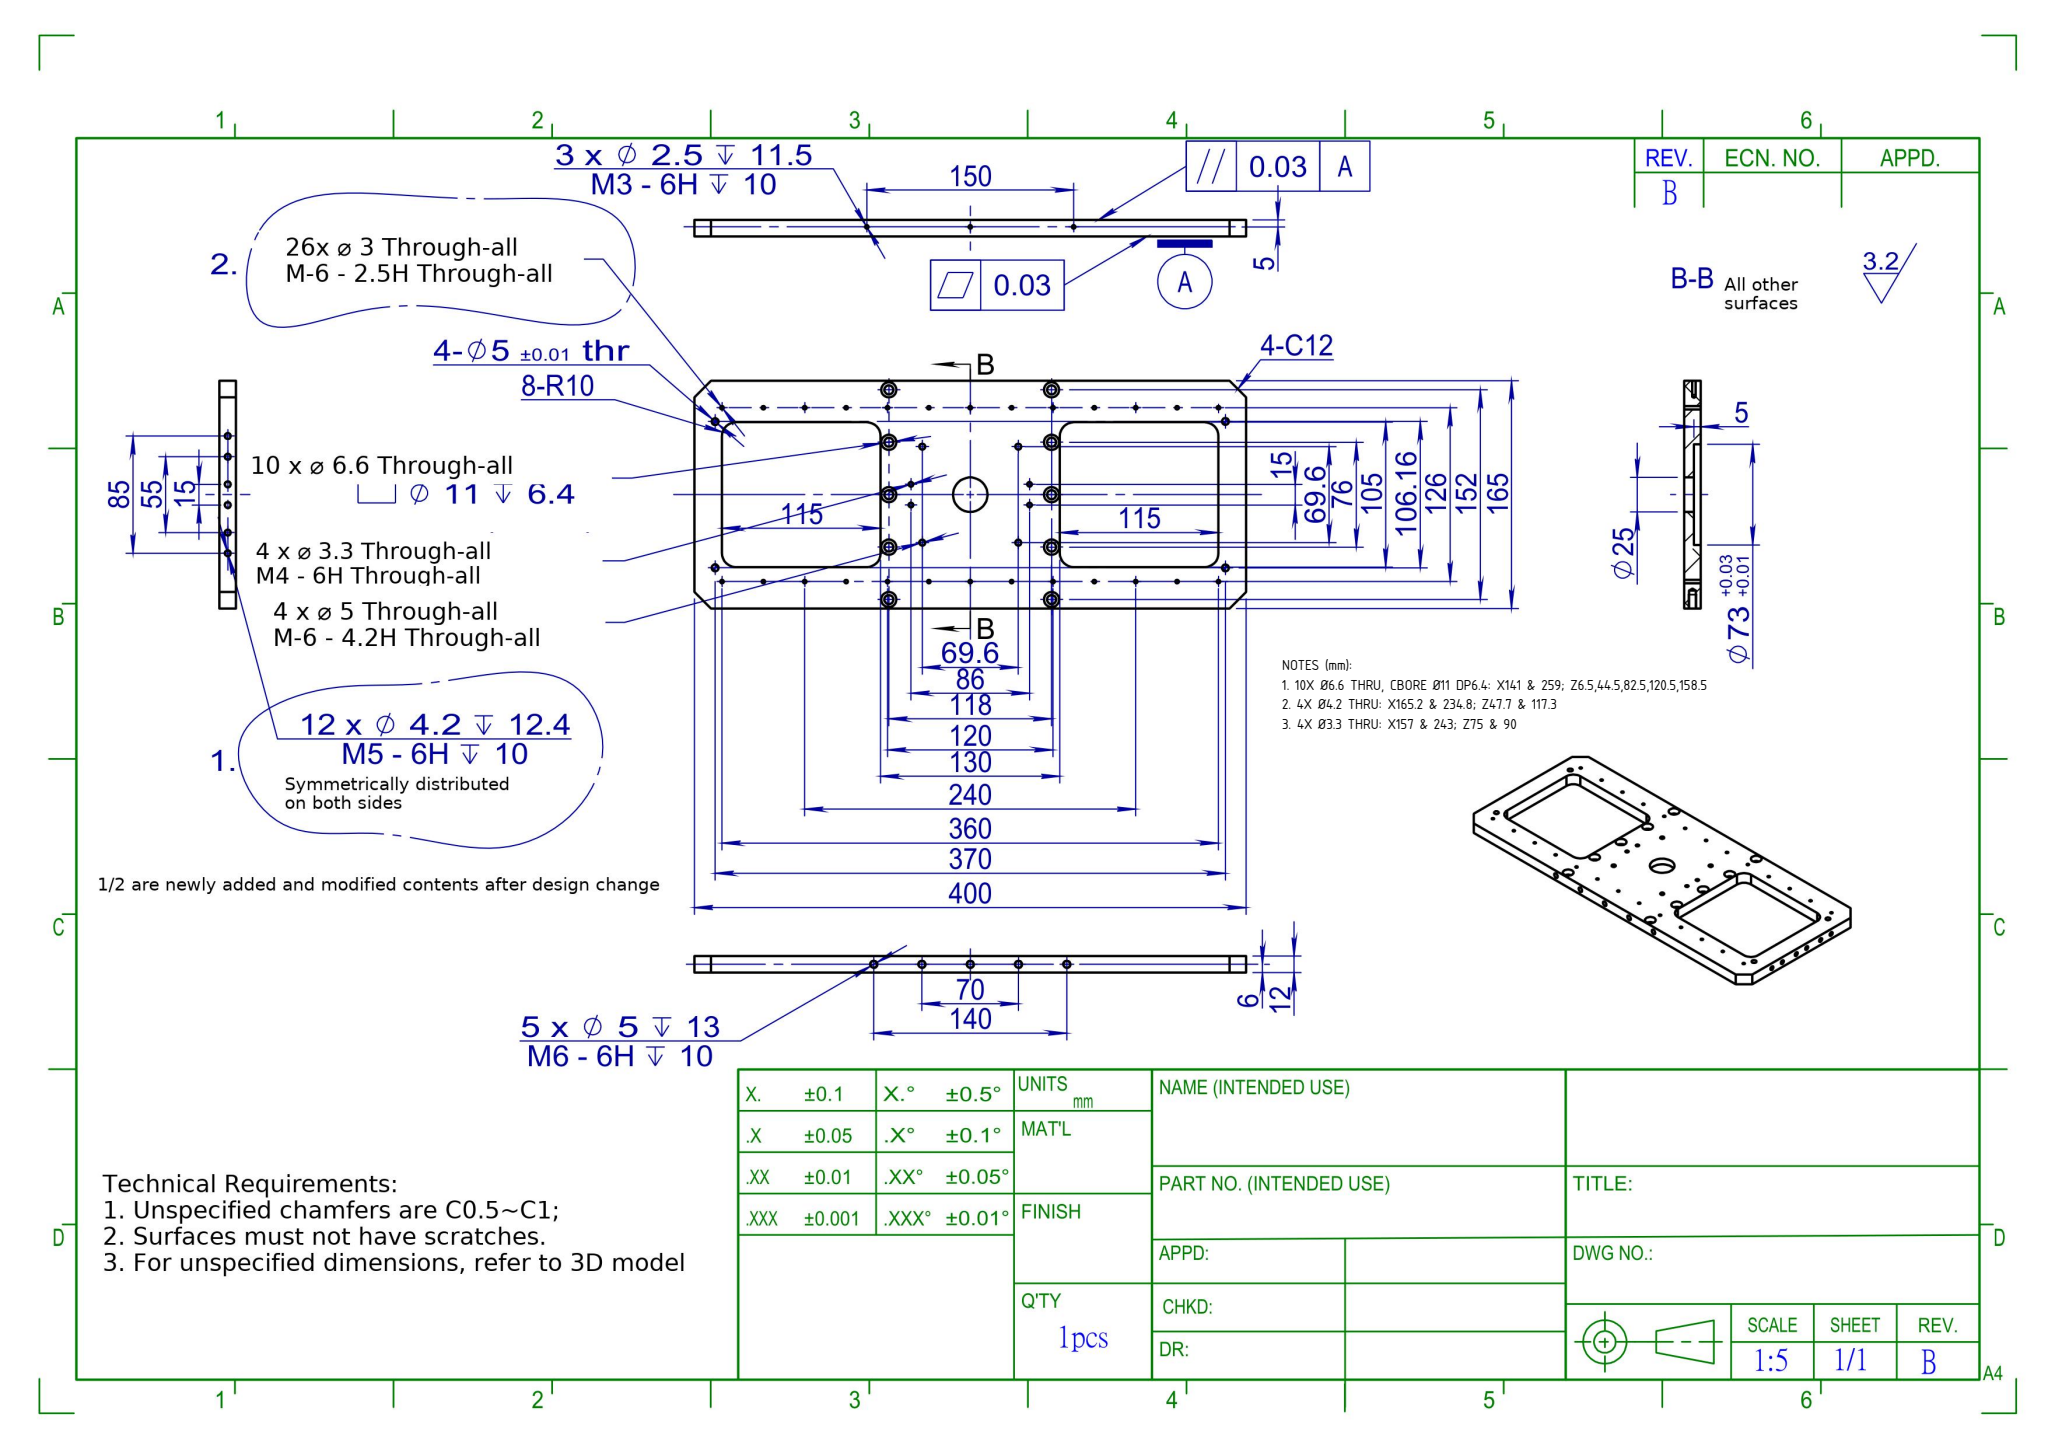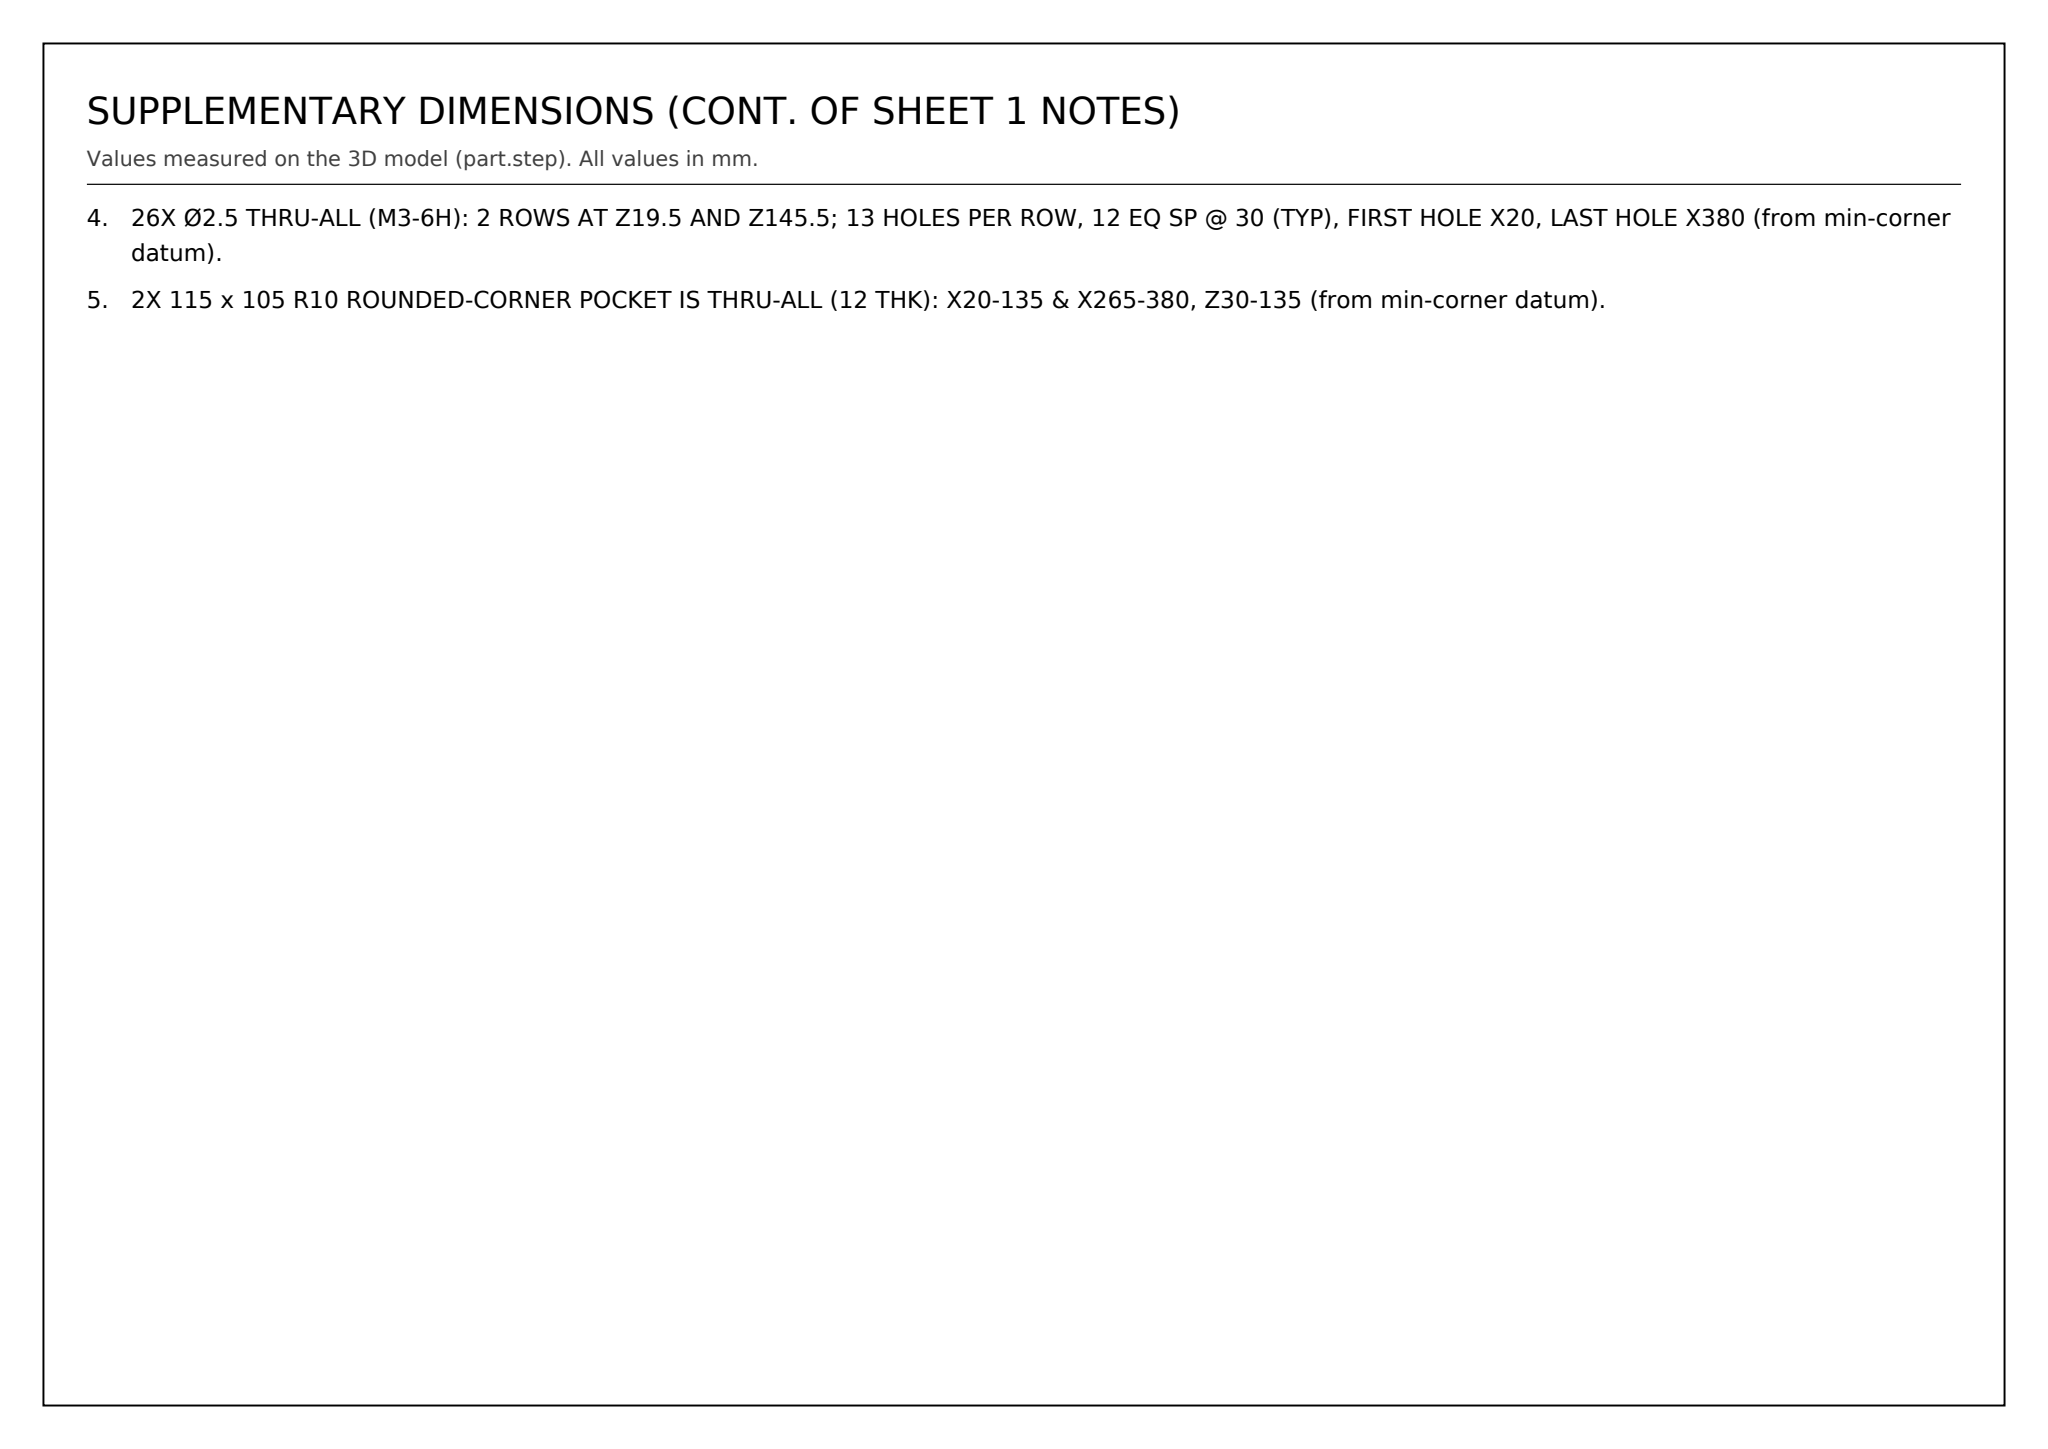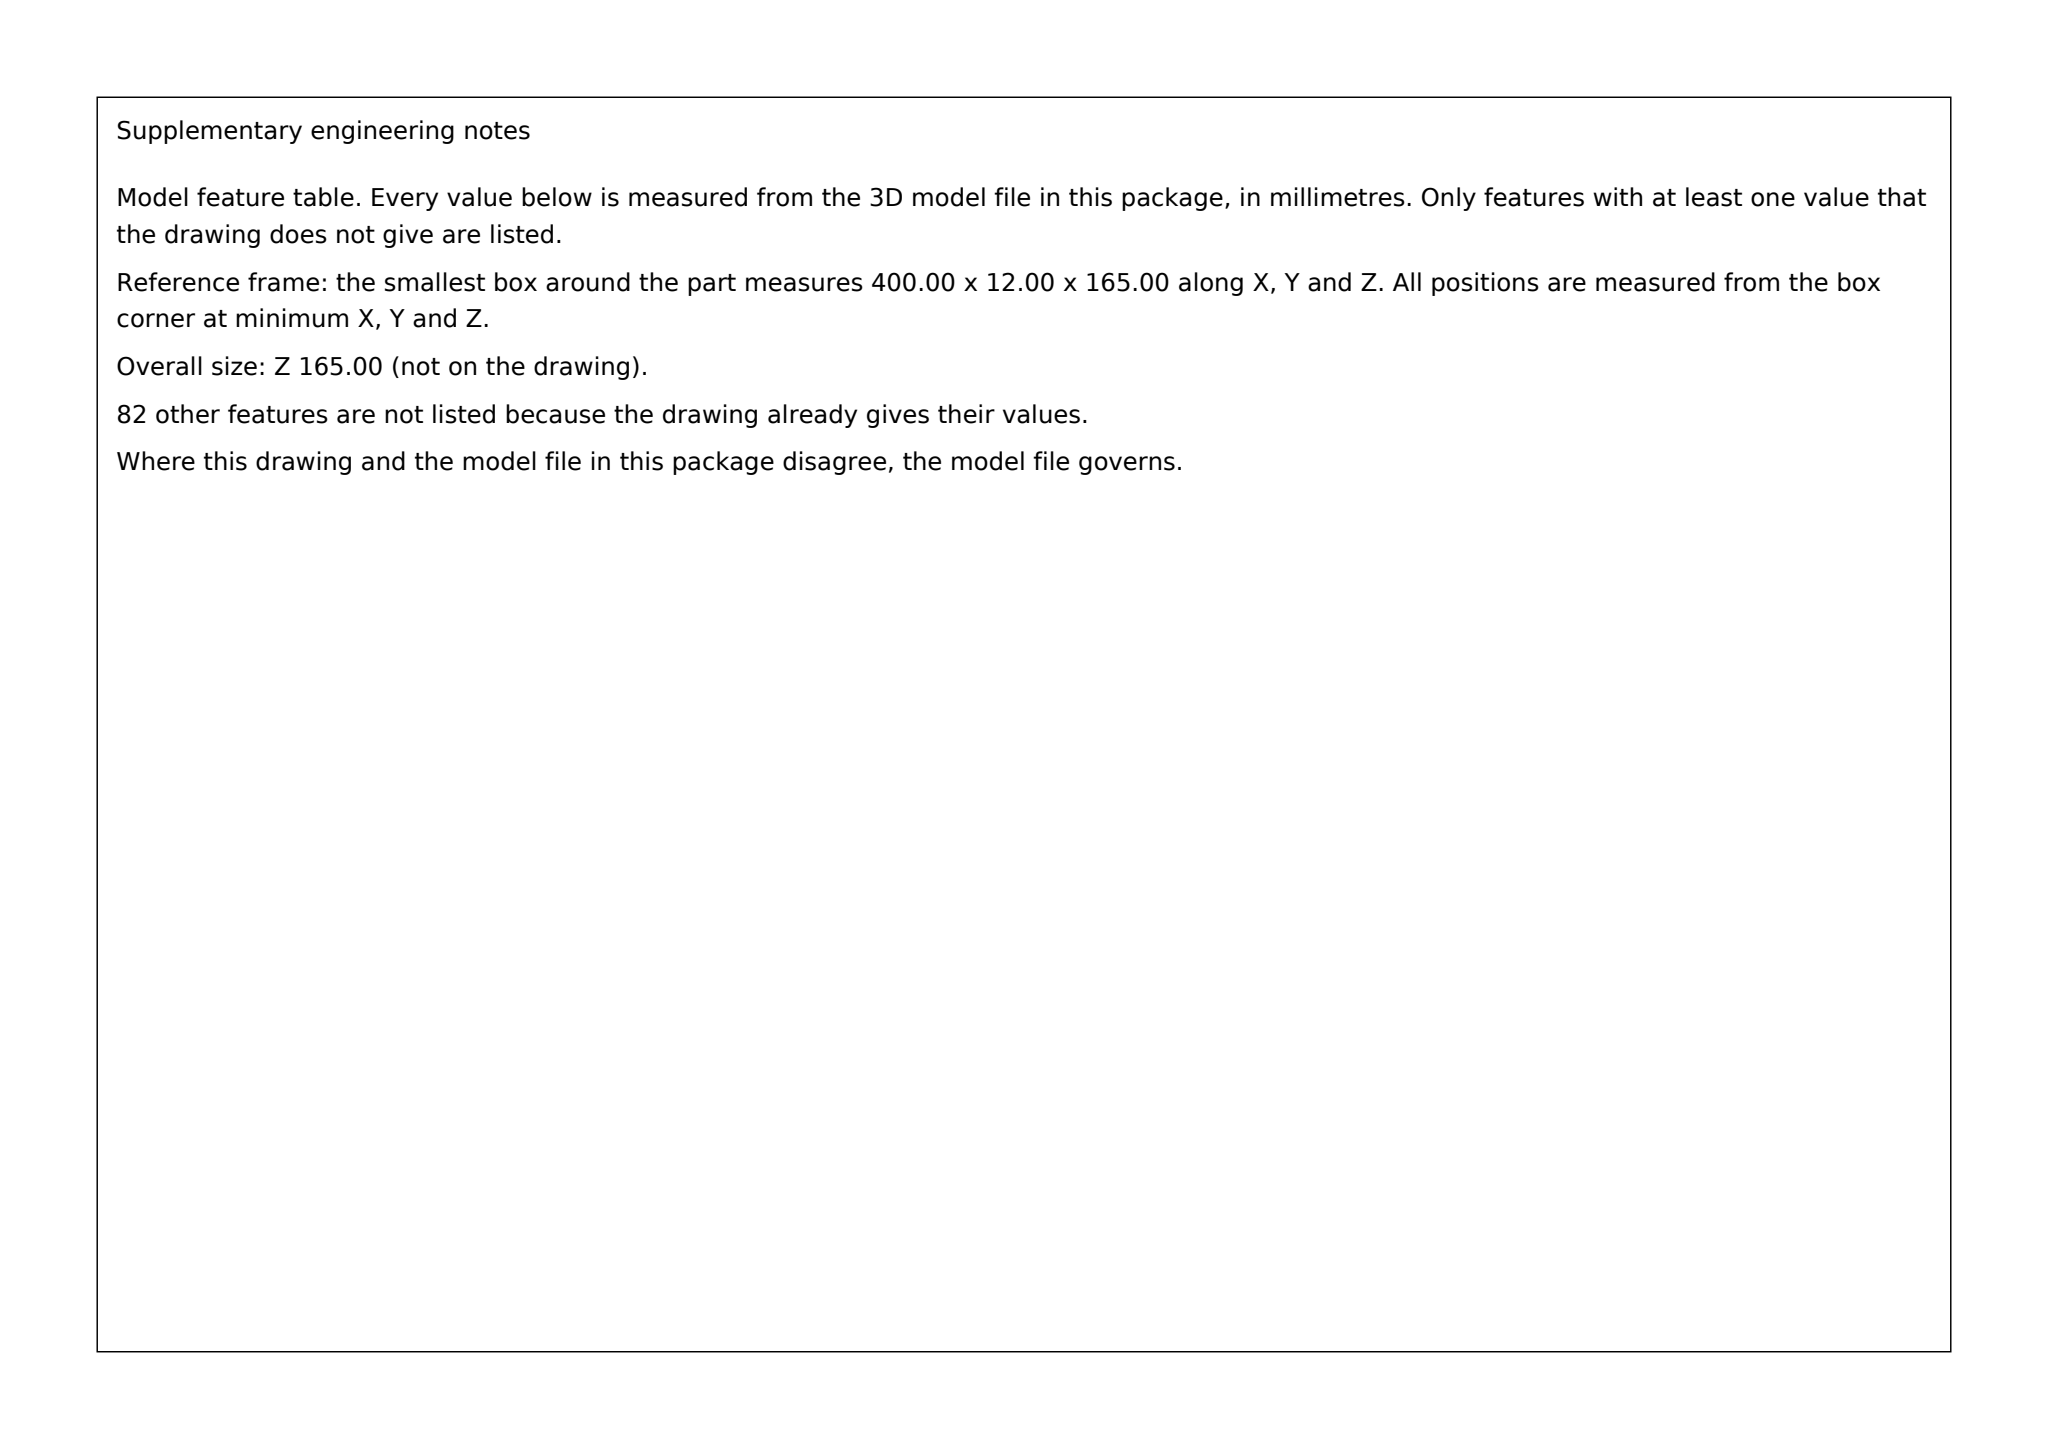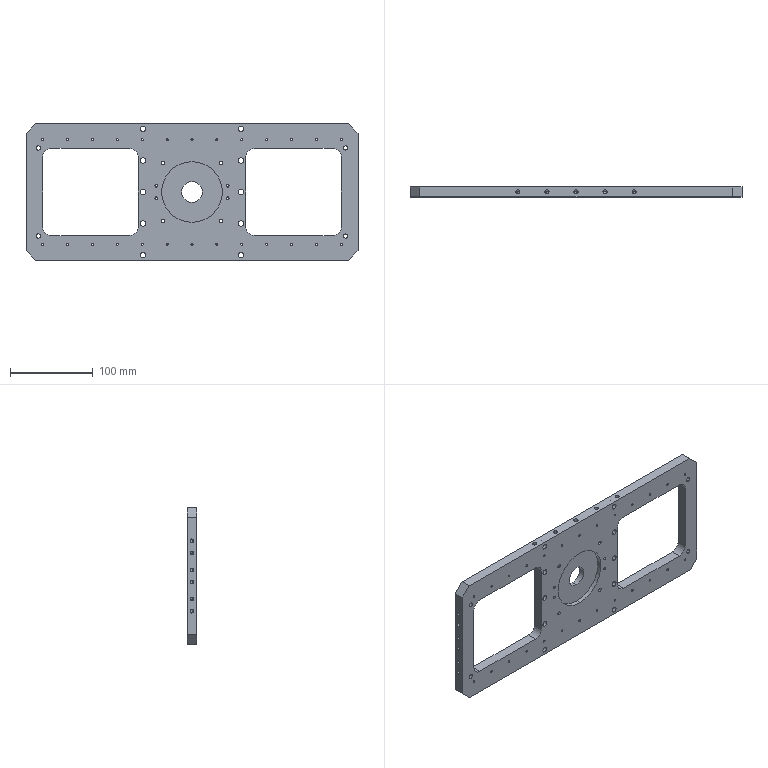Part | SolidWorks | mm | 1 solid | 237 faces | box 400 x 12 x 165 mm | volume 461264 mm3 | cylinder 168 | cone 40 | plane 29 | commonest cylinder face diameters 2.5 x58 4.2 x32 11 x20 6.6 x20 5 x18 3.3 x8 20 x8 73 x2
Drawing notes:
10X Ø6.6 THRU, CBORE Ø11 DP6.4: X141 & 259; Z6.5,44.5,82.5,120.5,158.5 | from the solid: [6.6,y,...,5.6] & [11.0,y,...,6.4] at x=141/259, z=6.5/44.5/82.5/120.5/158.5
4X Ø4.2 THRU: X165.2 & 234.8; Z47.7 & 117.3 | from the solid: [4.2,y,(165.2/234.8, z=47.7/117.3),12]
4X Ø3.3 THRU: X157 & 243; Z75 & 90 | from the solid: [3.3,y,(157/243, z=75/90),12]
26X Ø2.5 THRU-ALL (M3-6H): 2 ROWS AT Z19.5 AND Z145.5; 13 HOLES PER ROW, 12 EQ SP @ 30 (TYP), FIRST HOLE X20, LAST HOLE X380 (from min-corner datum). | from the solid: cylinders Ø2.5 axis y at z=19.5 & 145.5, x=20,50,80,110,140,170,200,230,260,290,320,350,380, from y0 to y12
2X 115 x 105 R10 ROUNDED-CORNER POCKET IS THRU-ALL (12 THK): X20-135 & X265-380, Z30-135 (from min-corner datum). | from the solid: axis_planes x=20,135,265,380 and z=30,135 each with y extent [0.0,12.0] equal to 12 mm plate thickness (bbox_xyz y=12)
build123d program:
from build123d import *

# Parameters (mm, degrees)
SKETCH1_W                                            = 400
SKETCH1_H                                            = 165
BOSS_EXTRUDE1_DEPTH                                  = 12
SKETCH2_R                                            = 12.5
CUT_EXTRUDE1_DEPTH                                   = 10
SKETCH3_R                                            = 36.5
CUT_EXTRUDE2_DEPTH                                   = 5
SKETCH4_W                                            = 115
SKETCH4_H                                            = 105
CUT_EXTRUDE3_DEPTH                                   = 217.68
FILLET1_R                                            = 10
FILLET1_OF_MIRROR1_R                                 = 10
CHAMFER1_SIZE                                        = 12
M5_TAPPED_HOLE1_AT_2_COUNT                           = 2
M5_TAPPED_HOLE1_AT_2_PITCH                           = 15
M6_HEX_SOCKET_HEAD_CAP_SCREW_COUNTERBORE_D           = 6.6
M6_HEX_SOCKET_HEAD_CAP_SCREW_COUNTERBORE_CBORE_D     = 11
M6_HEX_SOCKET_HEAD_CAP_SCREW_COUNTERBORE_CBORE_DEPTH = 6.4
LINEAR_PATTERN1_COUNT                                = 3
LINEAR_PATTERN1_PITCH                                = 38
LINEAR_PATTERN1_COL_COUNT                            = 3
LINEAR_PATTERN1_COL_PITCH                            = 38
MIRROR3_COPY_1_D                                     = 6.6
MIRROR3_COPY_1_CBORE_D                               = 11
MIRROR3_COPY_1_CBORE_DEPTH                           = 6.4
MIRROR3_COPY_2_D                                     = 6.6
MIRROR3_COPY_2_CBORE_D                               = 11
MIRROR3_COPY_2_CBORE_DEPTH                           = 6.4
MIRROR3_COPY_3_D                                     = 6.6
MIRROR3_COPY_3_CBORE_D                               = 11
MIRROR3_COPY_3_CBORE_DEPTH                           = 6.4
MIRROR3_COPY_4_D                                     = 6.6
MIRROR3_COPY_4_CBORE_D                               = 11
MIRROR3_COPY_4_CBORE_DEPTH                           = 6.4
M6_TAPPED_HOLE1_D                                    = 5
M6_TAPPED_HOLE1_DEPTH                                = 13
M6_TAPPED_HOLE1_TIP                                  = 1.502
SKETCH11_R                                           = 2.5
CUT_EXTRUDE4_DEPTH                                   = 217.68
M3_TAPPED_HOLE1_D                                    = 2.5
LINEAR_PATTERN2_COUNT                                = 4
LINEAR_PATTERN2_PITCH                                = 60
LINEAR_PATTERN2_COL_COUNT                            = 4
LINEAR_PATTERN2_COL_PITCH                            = 60
MIRROR5_COPY_1_D                                     = 2.5
MIRROR5_COPY_2_D                                     = 2.5
MIRROR5_COPY_3_D                                     = 2.5
MIRROR5_COPY_4_D                                     = 2.5
MIRROR5_COPY_5_D                                     = 2.5
MIRROR5_COPY_6_D                                     = 2.5
M5_TAPPED_HOLE2_D                                    = 4.2
M3_TAPPED_HOLE2_D                                    = 2.5
M3_TAPPED_HOLE2_DEPTH                                = 11.5
M3_TAPPED_HOLE2_TIP                                  = 0.7511
M4_TAPPED_HOLE1_D                                    = 3.3
M3_TAPPED_HOLE3_D                                    = 2.5
LINEAR_PATTERN3_COUNT                                = 4
LINEAR_PATTERN3_PITCH                                = 60
LINEAR_PATTERN3_COL_COUNT                            = 3
LINEAR_PATTERN3_COL_PITCH                            = 60
MIRROR6_COPY_1_D                                     = 2.5
MIRROR6_COPY_2_D                                     = 2.5
MIRROR6_COPY_3_D                                     = 2.5
MIRROR6_COPY_4_D                                     = 2.5
MIRROR6_COPY_5_D                                     = 2.5
LINEAR_PATTERN4_COUNT                                = 2
LINEAR_PATTERN4_PITCH                                = 35
LINEAR_PATTERN4_COL_COUNT                            = 2
LINEAR_PATTERN4_COL_PITCH                            = 35


with BuildPart() as part:
    # Sketch1 → Boss-Extrude1 (new body)
    with BuildSketch(Plane(origin=(0, 0, 0), x_dir=(1, 0, 0), z_dir=(0, 1, 0))):
        Rectangle(SKETCH1_W, SKETCH1_H)
    extrude(amount=BOSS_EXTRUDE1_DEPTH)

    # Sketch2 → Cut-Extrude1 (cut)
    with BuildSketch(Plane(origin=(0, 12, 0), x_dir=(1, 0, 0), z_dir=(0, 1, 0))):
        with Locations(Location((0, 0, 0), (0, 0, 270))):
            Circle(SKETCH2_R)
    extrude(amount=-CUT_EXTRUDE1_DEPTH, mode=Mode.SUBTRACT)

    # Sketch3 → Cut-Extrude2 (cut)
    with BuildSketch(Plane.XZ):
        with Locations(Location((0, 0, 0), (0, 0, 270))):
            Circle(SKETCH3_R)
    extrude(amount=-CUT_EXTRUDE2_DEPTH, mode=Mode.SUBTRACT)

    # Sketch4 → Cut-Extrude3 (cut, through all)
    with BuildSketch(Plane.XZ):
        with Locations((122.5, 0)):
            Rectangle(SKETCH4_W, SKETCH4_H)
    cut_extrude3 = extrude(amount=-CUT_EXTRUDE3_DEPTH, mode=Mode.SUBTRACT)

    # Fillet1
    fillet1_edges = [part.edges().sort_by_distance(p)[0] for p in [
        (65, 6, -52.5),
        (65, 6, 52.5),
        (180, 6, 52.5),
        (180, 6, -52.5),
    ]]
    fillet(fillet1_edges, radius=FILLET1_R)

    # Mirror1: Cut-Extrude3 across plane
    add(cut_extrude3.mirror(Plane(origin=(0, 0, 0), x_dir=(0, 0, 1), z_dir=(1, 0, 0))), mode=Mode.SUBTRACT)

    # Fillet1 of Mirror1
    fillet1_of_mirror1_edges = [part.edges().sort_by_distance(p)[0] for p in [
        (-65, 6, -52.5),
        (-65, 6, 52.5),
        (-180, 6, 52.5),
        (-180, 6, -52.5),
    ]]
    fillet(fillet1_of_mirror1_edges, radius=FILLET1_OF_MIRROR1_R)

    # Chamfer1
    chamfer1_edges = [part.edges().sort_by_distance(p)[0] for p in [
        (-200, 6, -82.5),
        (200, 6, -82.5),
        (200, 6, 82.5),
        (-200, 6, 82.5),
    ]]
    chamfer(chamfer1_edges, length=CHAMFER1_SIZE)

    # Sketch5 → M5 Tapped Hole1 (revolve, cut)
    with BuildSketch(Plane(origin=(200, 6, 7.5), x_dir=(0, 0, -1), z_dir=(0, 1, 0))):
        Polygon((0, 0), (0, 13.662), (2.1, 12.4), (2.1, 0), align=None)
    m5_tapped_hole1 = revolve(axis=Axis((206.35, 6, 7.5), (-1, 0, 0)), mode=Mode.SUBTRACT)

    # M5 Tapped Hole1 at 2: M5 Tapped Hole1 ×2
    with Locations(*[(0, 0, -i * M5_TAPPED_HOLE1_AT_2_PITCH) for i in range(1, M5_TAPPED_HOLE1_AT_2_COUNT)]):
        add(m5_tapped_hole1, mode=Mode.SUBTRACT)

    # Mirror2: M5 Tapped Hole1 across plane
    add(m5_tapped_hole1.mirror(Plane(origin=(0, 0, 0), x_dir=(0, 0, 1), z_dir=(1, 0, 0))), mode=Mode.SUBTRACT)

    # Mirror2 copy 1 sketch → Mirror2 copy 1 (revolve, cut)
    with BuildSketch(Plane(origin=(-200, 6, -7.5), x_dir=(0, 0, -1), z_dir=(0, 1, 0))):
        Polygon((0, 0), (0, -13.662), (2.1, -12.4), (2.1, 0), align=None)
    revolve(axis=Axis((-206.35, 6, -7.5), (-1, 0, 0)), mode=Mode.SUBTRACT)

    # M6 Hex Socket Head Cap Screw Counterbore (through all)
    with Locations(Plane(origin=(0, 12, 0), x_dir=(1, 0, 0), z_dir=(0, 1, 0))):
        with Locations((-59, 0)):
            m6_hex_socket_head_cap_screw_counterbore = CounterBoreHole(M6_HEX_SOCKET_HEAD_CAP_SCREW_COUNTERBORE_D / 2, M6_HEX_SOCKET_HEAD_CAP_SCREW_COUNTERBORE_CBORE_D / 2, M6_HEX_SOCKET_HEAD_CAP_SCREW_COUNTERBORE_CBORE_DEPTH)

    # Linear Pattern1: M6 Hex Socket Head Cap Screw Counterbore ×3
    with Locations(*[(0, 0, i * LINEAR_PATTERN1_PITCH) for i in range(1, LINEAR_PATTERN1_COUNT)]):
        add(m6_hex_socket_head_cap_screw_counterbore, mode=Mode.SUBTRACT)

    # Linear Pattern1 col: M6 Hex Socket Head Cap Screw Counterbore ×3
    with Locations(*[(0, 0, -i * LINEAR_PATTERN1_COL_PITCH) for i in range(1, LINEAR_PATTERN1_COL_COUNT)]):
        add(m6_hex_socket_head_cap_screw_counterbore, mode=Mode.SUBTRACT)

    # Mirror3: M6 Hex Socket Head Cap Screw Counterbore across plane
    add(m6_hex_socket_head_cap_screw_counterbore.mirror(Plane(origin=(0, 0, 0), x_dir=(0, 0, 1), z_dir=(1, 0, 0))), mode=Mode.SUBTRACT)

    # Mirror3 copy 1 (through all)
    with Locations(Plane(origin=(0, 12, 38), x_dir=(-1, 0, 0), z_dir=(0, 1, 0))):
        with Locations((-59, 0)):
            CounterBoreHole(MIRROR3_COPY_1_D / 2, MIRROR3_COPY_1_CBORE_D / 2, MIRROR3_COPY_1_CBORE_DEPTH)

    # Mirror3 copy 2 (through all)
    with Locations(Plane(origin=(0, 12, 76), x_dir=(-1, 0, 0), z_dir=(0, 1, 0))):
        with Locations((-59, 0)):
            CounterBoreHole(MIRROR3_COPY_2_D / 2, MIRROR3_COPY_2_CBORE_D / 2, MIRROR3_COPY_2_CBORE_DEPTH)

    # Mirror3 copy 3 (through all)
    with Locations(Plane(origin=(0, 12, -38), x_dir=(-1, 0, 0), z_dir=(0, 1, 0))):
        with Locations((-59, 0)):
            CounterBoreHole(MIRROR3_COPY_3_D / 2, MIRROR3_COPY_3_CBORE_D / 2, MIRROR3_COPY_3_CBORE_DEPTH)

    # Mirror3 copy 4 (through all)
    with Locations(Plane(origin=(0, 12, -76), x_dir=(-1, 0, 0), z_dir=(0, 1, 0))):
        with Locations((-59, 0)):
            CounterBoreHole(MIRROR3_COPY_4_D / 2, MIRROR3_COPY_4_CBORE_D / 2, MIRROR3_COPY_4_CBORE_DEPTH)

    # M6 Tapped Hole1
    with Locations(Plane.XY.offset(82.5)):
        with Locations((0, 6), (-35, 6), (-70, 6), (35, 6), (70, 6)):
            Hole(M6_TAPPED_HOLE1_D / 2, depth=M6_TAPPED_HOLE1_DEPTH)
            with Locations((0, 0, -(M6_TAPPED_HOLE1_DEPTH + M6_TAPPED_HOLE1_TIP / 2))):  # 118° drill point
                Cone(0, M6_TAPPED_HOLE1_D / 2, M6_TAPPED_HOLE1_TIP, mode=Mode.SUBTRACT)

    # Sketch11 → Cut-Extrude4 (cut, through all)
    with BuildSketch(Plane(origin=(0, 12, 0), x_dir=(1, 0, 0), z_dir=(0, 1, 0))):
        with Locations(Location((-185, 53, 0), (0, 0, 270))):
            Circle(SKETCH11_R)
        with Locations(Location((185, 53.078, 0), (0, 0, 270))):
            Circle(SKETCH11_R)
    cut_extrude4 = extrude(amount=-CUT_EXTRUDE4_DEPTH, mode=Mode.SUBTRACT)

    # Mirror4: Cut-Extrude4 across plane
    add(cut_extrude4.mirror(Plane.XY), mode=Mode.SUBTRACT)

    # M3 Tapped Hole1 (through all)
    with Locations(Plane(origin=(0, 12, 0), x_dir=(1, 0, 0), z_dir=(0, 1, 0))):
        with Locations((0, 63)):
            m3_tapped_hole1 = Hole(M3_TAPPED_HOLE1_D / 2)

    # Linear Pattern2: M3 Tapped Hole1 ×4
    with Locations(*[(-i * LINEAR_PATTERN2_PITCH, 0, 0) for i in range(1, LINEAR_PATTERN2_COUNT)]):
        add(m3_tapped_hole1, mode=Mode.SUBTRACT)

    # Linear Pattern2 col: M3 Tapped Hole1 ×4
    with Locations(*[(i * LINEAR_PATTERN2_COL_PITCH, 0, 0) for i in range(1, LINEAR_PATTERN2_COL_COUNT)]):
        add(m3_tapped_hole1, mode=Mode.SUBTRACT)

    # Mirror5: M3 Tapped Hole1 across plane
    add(m3_tapped_hole1.mirror(Plane.XY), mode=Mode.SUBTRACT)

    # Mirror5 copy 1 (through all)
    with Locations(Plane(origin=(-60, 12, 0), x_dir=(1, 0, 0), z_dir=(0, 1, 0))):
        with Locations((0, -63)):
            Hole(MIRROR5_COPY_1_D / 2)

    # Mirror5 copy 2 (through all)
    with Locations(Plane(origin=(-120, 12, 0), x_dir=(1, 0, 0), z_dir=(0, 1, 0))):
        with Locations((0, -63)):
            Hole(MIRROR5_COPY_2_D / 2)

    # Mirror5 copy 3 (through all)
    with Locations(Plane(origin=(-180, 12, 0), x_dir=(1, 0, 0), z_dir=(0, 1, 0))):
        with Locations((0, -63)):
            Hole(MIRROR5_COPY_3_D / 2)

    # Mirror5 copy 4 (through all)
    with Locations(Plane(origin=(60, 12, 0), x_dir=(1, 0, 0), z_dir=(0, 1, 0))):
        with Locations((0, -63)):
            Hole(MIRROR5_COPY_4_D / 2)

    # Mirror5 copy 5 (through all)
    with Locations(Plane(origin=(120, 12, 0), x_dir=(1, 0, 0), z_dir=(0, 1, 0))):
        with Locations((0, -63)):
            Hole(MIRROR5_COPY_5_D / 2)

    # Mirror5 copy 6 (through all)
    with Locations(Plane(origin=(180, 12, 0), x_dir=(1, 0, 0), z_dir=(0, 1, 0))):
        with Locations((0, -63)):
            Hole(MIRROR5_COPY_6_D / 2)

    # M5 Tapped Hole2 (through all)
    with Locations(Plane(origin=(0, 0, 0), x_dir=(-1, 0, 0), z_dir=(0, -1, 0))):
        with Locations((34.8, -34.8), (-34.8, -34.8), (34.8, 34.8), (-34.8, 34.8)):
            Hole(M5_TAPPED_HOLE2_D / 2)

    # M3 Tapped Hole2
    with Locations(Plane(origin=(0, 0, -82.5), x_dir=(-1, 0, 0), z_dir=(0, 0, -1))):
        with Locations((-75, 5), (0, 5), (75, 5)):
            Hole(M3_TAPPED_HOLE2_D / 2, depth=M3_TAPPED_HOLE2_DEPTH)
            with Locations((0, 0, -(M3_TAPPED_HOLE2_DEPTH + M3_TAPPED_HOLE2_TIP / 2))):  # 118° drill point
                Cone(0, M3_TAPPED_HOLE2_D / 2, M3_TAPPED_HOLE2_TIP, mode=Mode.SUBTRACT)

    # M4 Tapped Hole1 (through all)
    with Locations(Plane(origin=(0, 12, 0), x_dir=(1, 0, 0), z_dir=(0, 1, 0))):
        with Locations((-43, 7.5), (-43, -7.5), (43, 7.5), (43, -7.5)):
            Hole(M4_TAPPED_HOLE1_D / 2)

    # M3 Tapped Hole3 (through all)
    with Locations(Plane(origin=(0, 12, 0), x_dir=(1, 0, 0), z_dir=(0, 1, 0))):
        with Locations((30, -63)):
            m3_tapped_hole3 = Hole(M3_TAPPED_HOLE3_D / 2)

    # Linear Pattern3: M3 Tapped Hole3 ×4
    with Locations(*[(-i * LINEAR_PATTERN3_PITCH, 0, 0) for i in range(1, LINEAR_PATTERN3_COUNT)]):
        add(m3_tapped_hole3, mode=Mode.SUBTRACT)

    # Linear Pattern3 col: M3 Tapped Hole3 ×3
    with Locations(*[(i * LINEAR_PATTERN3_COL_PITCH, 0, 0) for i in range(1, LINEAR_PATTERN3_COL_COUNT)]):
        add(m3_tapped_hole3, mode=Mode.SUBTRACT)

    # Mirror6: M3 Tapped Hole3 across plane
    add(m3_tapped_hole3.mirror(Plane.XY), mode=Mode.SUBTRACT)

    # Mirror6 copy 1 (through all)
    with Locations(Plane(origin=(-60, 12, 0), x_dir=(1, 0, 0), z_dir=(0, 1, 0))):
        with Locations((30, 63)):
            Hole(MIRROR6_COPY_1_D / 2)

    # Mirror6 copy 2 (through all)
    with Locations(Plane(origin=(-120, 12, 0), x_dir=(1, 0, 0), z_dir=(0, 1, 0))):
        with Locations((30, 63)):
            Hole(MIRROR6_COPY_2_D / 2)

    # Mirror6 copy 3 (through all)
    with Locations(Plane(origin=(-180, 12, 0), x_dir=(1, 0, 0), z_dir=(0, 1, 0))):
        with Locations((30, 63)):
            Hole(MIRROR6_COPY_3_D / 2)

    # Mirror6 copy 4 (through all)
    with Locations(Plane(origin=(60, 12, 0), x_dir=(1, 0, 0), z_dir=(0, 1, 0))):
        with Locations((30, 63)):
            Hole(MIRROR6_COPY_4_D / 2)

    # Mirror6 copy 5 (through all)
    with Locations(Plane(origin=(120, 12, 0), x_dir=(1, 0, 0), z_dir=(0, 1, 0))):
        with Locations((30, 63)):
            Hole(MIRROR6_COPY_5_D / 2)

    # Linear Pattern4: M5 Tapped Hole1 ×2
    with Locations(*[(0, 0, -i * LINEAR_PATTERN4_PITCH) for i in range(1, LINEAR_PATTERN4_COUNT)]):
        add(m5_tapped_hole1, mode=Mode.SUBTRACT)

    # Linear Pattern4 copy 1 sketch → Linear Pattern4 copy 1 (revolve, cut)
    with BuildSketch(Plane(origin=(200, 6, -42.5), x_dir=(0, 0, -1), z_dir=(0, 1, 0))):
        Polygon((0, 0), (0, 13.662), (2.1, 12.4), (2.1, 0), align=None)
    revolve(axis=Axis((206.35, 6, -42.5), (-1, 0, 0)), mode=Mode.SUBTRACT)

    # Linear Pattern4 col: M5 Tapped Hole1 ×2
    with Locations(*[(0, 0, i * LINEAR_PATTERN4_COL_PITCH) for i in range(1, LINEAR_PATTERN4_COL_COUNT)]):
        add(m5_tapped_hole1, mode=Mode.SUBTRACT)

    # Linear Pattern4 col copy 1 sketch → Linear Pattern4 col copy 1 (revolve, cut)
    with BuildSketch(Plane(origin=(200, 6, 27.5), x_dir=(0, 0, -1), z_dir=(0, 1, 0))):
        Polygon((0, 0), (0, 13.662), (2.1, 12.4), (2.1, 0), align=None)
    revolve(axis=Axis((206.35, 6, 27.5), (-1, 0, 0)), mode=Mode.SUBTRACT)

    # Mirror7 copy 1 sketch → Mirror7 copy 1 (revolve, cut)
    with BuildSketch(Plane(origin=(-200, 6, -27.5), x_dir=(0, 0, -1), z_dir=(0, 1, 0))):
        Polygon((0, 0), (0, -13.662), (2.1, -12.4), (2.1, 0), align=None)
    revolve(axis=Axis((-206.35, 6, -27.5), (-1, 0, 0)), mode=Mode.SUBTRACT)

    # Mirror7 copy 2 sketch → Mirror7 copy 2 (revolve, cut)
    with BuildSketch(Plane(origin=(-200, 6, -42.5), x_dir=(0, 0, -1), z_dir=(0, 1, 0))):
        Polygon((0, 0), (0, -13.662), (2.1, -12.4), (2.1, 0), align=None)
    revolve(axis=Axis((-206.35, 6, -42.5), (-1, 0, 0)), mode=Mode.SUBTRACT)

    # Mirror7 copy 3 sketch → Mirror7 copy 3 (revolve, cut)
    with BuildSketch(Plane(origin=(-200, 6, 42.5), x_dir=(0, 0, -1), z_dir=(0, 1, 0))):
        Polygon((0, 0), (0, -13.662), (2.1, -12.4), (2.1, 0), align=None)
    revolve(axis=Axis((-206.35, 6, 42.5), (-1, 0, 0)), mode=Mode.SUBTRACT)

    # Mirror7 copy 4 sketch → Mirror7 copy 4 (revolve, cut)
    with BuildSketch(Plane(origin=(-200, 6, 27.5), x_dir=(0, 0, -1), z_dir=(0, 1, 0))):
        Polygon((0, 0), (0, -13.662), (2.1, -12.4), (2.1, 0), align=None)
    revolve(axis=Axis((-206.35, 6, 27.5), (-1, 0, 0)), mode=Mode.SUBTRACT)

    # Mirror7 copy 5 sketch → Mirror7 copy 5 (revolve, cut)
    with BuildSketch(Plane(origin=(-200, 6, 7.5), x_dir=(0, 0, -1), z_dir=(0, 1, 0))):
        Polygon((0, 0), (0, -13.662), (2.1, -12.4), (2.1, 0), align=None)
    revolve(axis=Axis((-206.35, 6, 7.5), (-1, 0, 0)), mode=Mode.SUBTRACT)

    # Mirror7 copy 6 sketch → Mirror7 copy 6 (revolve, cut)
    with BuildSketch(Plane(origin=(-200, 6, -7.5), x_dir=(0, 0, -1), z_dir=(0, 1, 0))):
        Polygon((0, 0), (0, -13.662), (2.1, -12.4), (2.1, 0), align=None)
    revolve(axis=Axis((-206.35, 6, -7.5), (-1, 0, 0)), mode=Mode.SUBTRACT)


solid = part.part